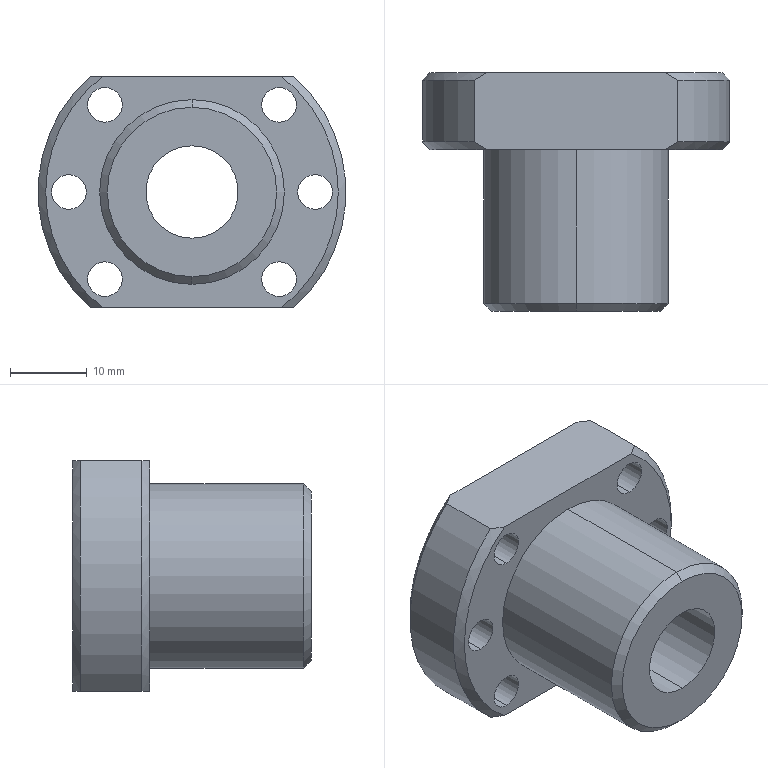Component | SolidWorks | SFS01205Nut--1 | 1 solid | 29 faces | box 40 x 31 x 30 mm | volume 15688 mm3 | cylinder 18 | cone 6 | plane 5 | commonest cylinder face diameters 4.5 x12 24 x2 12 x2 40 x2
build123d program:
from build123d import *

# Parameters (mm, degrees)
CUT_EXTRUDE1_DEPTH = 42.964
SKETCH3_R          = 2.25
CUT_EXTRUDE2_DEPTH = 40.825
CHAMFER1_SIZE      = 1


with BuildPart() as part:
    # Sketch1 → Revolve1 (revolve)
    with BuildSketch(Plane(origin=(0, 0, 0), x_dir=(1, 0, 0), z_dir=(0, 1, 0))):
        Polygon((-31, 6), (-31, 20), (-21, 20), (-21, 12), (0, 12), (0, 6), align=None)
    revolve(axis=Axis((0, 0, 0), (-1, 0, 0)))

    # Sketch2 → Cut-Extrude1 (cut, symmetric)
    with BuildSketch(Plane.ZY.offset(31)):
        Polygon((15, 119.751), (15, 13.229), (15, -13.229), (15, -119.751), (228.045, -119.751), (228.045, 119.751), align=None)
    cut_extrude1 = extrude(amount=CUT_EXTRUDE1_DEPTH, both=True, mode=Mode.SUBTRACT)

    # Mirror1: Cut-Extrude1 across plane
    add(cut_extrude1.mirror(Plane.XY), mode=Mode.SUBTRACT)

    # Sketch3 → Cut-Extrude2 (cut, through all)
    with BuildSketch(Plane.ZY.offset(31)):
        with Locations((-11.314, 11.314)):
            Circle(SKETCH3_R)
        with Locations(Location((11.314, 11.314, 0), (0, 0, 180))):
            Circle(SKETCH3_R)
        with Locations((0, 16)):
            Circle(SKETCH3_R)
        with Locations(Location((0, -16, 0), (0, 0, 180))):
            Circle(SKETCH3_R)
        with Locations((11.314, -11.314)):
            Circle(SKETCH3_R)
        with Locations(Location((-11.314, -11.314, 0), (0, 0, 180))):
            Circle(SKETCH3_R)
    extrude(amount=-CUT_EXTRUDE2_DEPTH, mode=Mode.SUBTRACT)

    # Chamfer1
    chamfer1_edges = [part.edges().sort_by_distance(p)[0] for p in [
        (-21, -20, 0),
        (-31, -20, 0),
        (-21, 20, 0),
        (-31, 20, 0),
        (0, 0, 12),
    ]]
    chamfer(chamfer1_edges, length=CHAMFER1_SIZE)


solid = part.part

# Placed as in the assembly
solid = solid.moved(Location((-109.352, -196.452, -272.475), (0, 0, -90)))
STEP:
#1=COLOUR_RGB('',0.7922,0.8196,0.9333);
#2=FILL_AREA_STYLE_COLOUR('',#1);
#3=FILL_AREA_STYLE('',(#2));
#4=SURFACE_STYLE_FILL_AREA(#3);
#5=SURFACE_SIDE_STYLE('',(#4));
#6=SURFACE_STYLE_USAGE(.BOTH.,#5);
#7=PRESENTATION_STYLE_ASSIGNMENT((#6));
#8=CARTESIAN_POINT('',(-4.305,-7.734,-11.16));
#9=VERTEX_POINT('',#8);
#10=CARTESIAN_POINT('',(-4.305,-7.734,-10.294));
#11=VERTEX_POINT('',#10);
#12=CARTESIAN_POINT('',(-4.305,-7.734,-10.727));
#13=DIRECTION('',(-0.,-1.,0.));
#14=DIRECTION('',(-0.,0.,-1.));
#15=AXIS2_PLACEMENT_3D('',#12,#13,#14);
#16=CIRCLE('',#15,0.4331);
#17=EDGE_CURVE('',#9,#11,#16,.T.);
#18=ORIENTED_EDGE('',*,*,#17,.F.);
#19=CARTESIAN_POINT('',(-4.305,-7.695,-11.2));
#20=VERTEX_POINT('',#19);
#21=CARTESIAN_POINT('',(-4.305,-7.734,-11.16));
#22=DIRECTION('',(-0.,0.7071,-0.7071));
#23=VECTOR('',#22,39.37);
#24=LINE('',#21,#23);
#25=EDGE_CURVE('',#9,#20,#24,.T.);
#26=ORIENTED_EDGE('',*,*,#25,.T.);
#27=CARTESIAN_POINT('',(-4.305,-7.695,-10.255));
#28=VERTEX_POINT('',#27);
#29=CARTESIAN_POINT('',(-4.305,-7.695,-10.727));
#30=DIRECTION('',(0.,1.,-0.));
#31=DIRECTION('',(-0.,0.,-1.));
#32=AXIS2_PLACEMENT_3D('',#29,#30,#31);
#33=CIRCLE('',#32,0.4724);
#34=EDGE_CURVE('',#28,#20,#33,.T.);
#35=ORIENTED_EDGE('',*,*,#34,.F.);
#36=CARTESIAN_POINT('',(-4.305,-7.734,-10.294));
#37=DIRECTION('',(0.,0.7071,0.7071));
#38=VECTOR('',#37,39.37);
#39=LINE('',#36,#38);
#40=EDGE_CURVE('',#11,#28,#39,.T.);
#41=ORIENTED_EDGE('',*,*,#40,.F.);
#42=EDGE_LOOP('',(#18,#26,#35,#41));
#43=FACE_OUTER_BOUND('',#42,.T.);
#44=CARTESIAN_POINT('',(-4.305,-7.734,-10.727));
#45=DIRECTION('',(0.,1.,-0.));
#46=DIRECTION('',(0.,0.,1.));
#47=AXIS2_PLACEMENT_3D('',#44,#45,#46);
#48=CONICAL_SURFACE('',#47,0.4331,0.7854);
#49=ADVANCED_FACE('',(#43),#48,.T.);
#50=CARTESIAN_POINT('',(-4.751,-6.908,-11.084));
#51=VERTEX_POINT('',#50);
#52=CARTESIAN_POINT('',(-4.751,-6.908,-11.261));
#53=VERTEX_POINT('',#52);
#54=CARTESIAN_POINT('',(-4.751,-6.908,-11.173));
#55=DIRECTION('',(-0.,-1.,0.));
#56=DIRECTION('',(-0.,0.,-1.));
#57=AXIS2_PLACEMENT_3D('',#54,#55,#56);
#58=CIRCLE('',#57,0.08858);
#59=EDGE_CURVE('',#51,#53,#58,.T.);
#60=ORIENTED_EDGE('',*,*,#59,.T.);
#61=CARTESIAN_POINT('',(-4.751,-6.514,-11.261));
#62=VERTEX_POINT('',#61);
#63=CARTESIAN_POINT('',(-4.751,-7.734,-11.261));
#64=DIRECTION('',(0.,1.,-0.));
#65=VECTOR('',#64,39.37);
#66=LINE('',#63,#65);
#67=EDGE_CURVE('',#53,#62,#66,.T.);
#68=ORIENTED_EDGE('',*,*,#67,.T.);
#69=CARTESIAN_POINT('',(-4.751,-6.514,-11.084));
#70=VERTEX_POINT('',#69);
#71=CARTESIAN_POINT('',(-4.751,-6.514,-11.173));
#72=DIRECTION('',(0.,1.,-0.));
#73=DIRECTION('',(-0.,0.,-1.));
#74=AXIS2_PLACEMENT_3D('',#71,#72,#73);
#75=CIRCLE('',#74,0.08858);
#76=EDGE_CURVE('',#62,#70,#75,.T.);
#77=ORIENTED_EDGE('',*,*,#76,.T.);
#78=CARTESIAN_POINT('',(-4.751,-7.734,-11.084));
#79=DIRECTION('',(0.,1.,-0.));
#80=VECTOR('',#79,39.37);
#81=LINE('',#78,#80);
#82=EDGE_CURVE('',#51,#70,#81,.T.);
#83=ORIENTED_EDGE('',*,*,#82,.F.);
#84=EDGE_LOOP('',(#60,#68,#77,#83));
#85=FACE_OUTER_BOUND('',#84,.T.);
#86=CARTESIAN_POINT('',(-4.751,-7.734,-11.173));
#87=DIRECTION('',(0.,1.,-0.));
#88=DIRECTION('',(0.,0.,1.));
#89=AXIS2_PLACEMENT_3D('',#86,#87,#88);
#90=CYLINDRICAL_SURFACE('',#89,0.08858);
#91=ADVANCED_FACE('',(#85),#90,.F.);
#92=CARTESIAN_POINT('',(-4.751,-6.908,-10.193));
#93=VERTEX_POINT('',#92);
#94=CARTESIAN_POINT('',(-4.751,-6.908,-10.371));
#95=VERTEX_POINT('',#94);
#96=CARTESIAN_POINT('',(-4.751,-6.908,-10.282));
#97=DIRECTION('',(-0.,-1.,0.));
#98=DIRECTION('',(-0.,0.,-1.));
#99=AXIS2_PLACEMENT_3D('',#96,#97,#98);
#100=CIRCLE('',#99,0.08858);
#101=EDGE_CURVE('',#93,#95,#100,.T.);
#102=ORIENTED_EDGE('',*,*,#101,.T.);
#103=CARTESIAN_POINT('',(-4.751,-6.514,-10.371));
#104=VERTEX_POINT('',#103);
#105=CARTESIAN_POINT('',(-4.751,-7.734,-10.371));
#106=DIRECTION('',(0.,1.,-0.));
#107=VECTOR('',#106,39.37);
#108=LINE('',#105,#107);
#109=EDGE_CURVE('',#95,#104,#108,.T.);
#110=ORIENTED_EDGE('',*,*,#109,.T.);
#111=CARTESIAN_POINT('',(-4.751,-6.514,-10.193));
#112=VERTEX_POINT('',#111);
#113=CARTESIAN_POINT('',(-4.751,-6.514,-10.282));
#114=DIRECTION('',(0.,1.,-0.));
#115=DIRECTION('',(0.,0.,1.));
#116=AXIS2_PLACEMENT_3D('',#113,#114,#115);
#117=CIRCLE('',#116,0.08858);
#118=EDGE_CURVE('',#104,#112,#117,.T.);
#119=ORIENTED_EDGE('',*,*,#118,.T.);
#120=CARTESIAN_POINT('',(-4.751,-7.734,-10.193));
#121=DIRECTION('',(0.,1.,-0.));
#122=VECTOR('',#121,39.37);
#123=LINE('',#120,#122);
#124=EDGE_CURVE('',#93,#112,#123,.T.);
#125=ORIENTED_EDGE('',*,*,#124,.F.);
#126=EDGE_LOOP('',(#102,#110,#119,#125));
#127=FACE_OUTER_BOUND('',#126,.T.);
#128=CARTESIAN_POINT('',(-4.751,-7.734,-10.282));
#129=DIRECTION('',(0.,1.,-0.));
#130=DIRECTION('',(0.,0.,1.));
#131=AXIS2_PLACEMENT_3D('',#128,#129,#130);
#132=CYLINDRICAL_SURFACE('',#131,0.08858);
#133=ADVANCED_FACE('',(#127),#132,.F.);
#134=CARTESIAN_POINT('',(-4.935,-6.908,-10.639));
#135=VERTEX_POINT('',#134);
#136=CARTESIAN_POINT('',(-4.935,-6.908,-10.816));
#137=VERTEX_POINT('',#136);
#138=CARTESIAN_POINT('',(-4.935,-6.908,-10.727));
#139=DIRECTION('',(-0.,-1.,0.));
#140=DIRECTION('',(-0.,0.,-1.));
#141=AXIS2_PLACEMENT_3D('',#138,#139,#140);
#142=CIRCLE('',#141,0.08858);
#143=EDGE_CURVE('',#135,#137,#142,.T.);
#144=ORIENTED_EDGE('',*,*,#143,.T.);
#145=CARTESIAN_POINT('',(-4.935,-6.514,-10.816));
#146=VERTEX_POINT('',#145);
#147=CARTESIAN_POINT('',(-4.935,-7.734,-10.816));
#148=DIRECTION('',(0.,1.,-0.));
#149=VECTOR('',#148,39.37);
#150=LINE('',#147,#149);
#151=EDGE_CURVE('',#137,#146,#150,.T.);
#152=ORIENTED_EDGE('',*,*,#151,.T.);
#153=CARTESIAN_POINT('',(-4.935,-6.514,-10.639));
#154=VERTEX_POINT('',#153);
#155=CARTESIAN_POINT('',(-4.935,-6.514,-10.727));
#156=DIRECTION('',(0.,1.,-0.));
#157=DIRECTION('',(-0.,0.,-1.));
#158=AXIS2_PLACEMENT_3D('',#155,#156,#157);
#159=CIRCLE('',#158,0.08858);
#160=EDGE_CURVE('',#146,#154,#159,.T.);
#161=ORIENTED_EDGE('',*,*,#160,.T.);
#162=CARTESIAN_POINT('',(-4.935,-7.734,-10.639));
#163=DIRECTION('',(0.,1.,-0.));
#164=VECTOR('',#163,39.37);
#165=LINE('',#162,#164);
#166=EDGE_CURVE('',#135,#154,#165,.T.);
#167=ORIENTED_EDGE('',*,*,#166,.F.);
#168=EDGE_LOOP('',(#144,#152,#161,#167));
#169=FACE_OUTER_BOUND('',#168,.T.);
#170=CARTESIAN_POINT('',(-4.935,-7.734,-10.727));
#171=DIRECTION('',(0.,1.,-0.));
#172=DIRECTION('',(0.,0.,1.));
#173=AXIS2_PLACEMENT_3D('',#170,#171,#172);
#174=CYLINDRICAL_SURFACE('',#173,0.08858);
#175=ADVANCED_FACE('',(#169),#174,.F.);
#176=CARTESIAN_POINT('',(-3.675,-6.908,-10.639));
#177=VERTEX_POINT('',#176);
#178=CARTESIAN_POINT('',(-3.675,-6.908,-10.816));
#179=VERTEX_POINT('',#178);
#180=CARTESIAN_POINT('',(-3.675,-6.908,-10.727));
#181=DIRECTION('',(-0.,-1.,0.));
#182=DIRECTION('',(-0.,0.,-1.));
#183=AXIS2_PLACEMENT_3D('',#180,#181,#182);
#184=CIRCLE('',#183,0.08858);
#185=EDGE_CURVE('',#177,#179,#184,.T.);
#186=ORIENTED_EDGE('',*,*,#185,.T.);
#187=CARTESIAN_POINT('',(-3.675,-6.514,-10.816));
#188=VERTEX_POINT('',#187);
#189=CARTESIAN_POINT('',(-3.675,-7.734,-10.816));
#190=DIRECTION('',(0.,1.,-0.));
#191=VECTOR('',#190,39.37);
#192=LINE('',#189,#191);
#193=EDGE_CURVE('',#179,#188,#192,.T.);
#194=ORIENTED_EDGE('',*,*,#193,.T.);
#195=CARTESIAN_POINT('',(-3.675,-6.514,-10.639));
#196=VERTEX_POINT('',#195);
#197=CARTESIAN_POINT('',(-3.675,-6.514,-10.727));
#198=DIRECTION('',(0.,1.,-0.));
#199=DIRECTION('',(0.,0.,1.));
#200=AXIS2_PLACEMENT_3D('',#197,#198,#199);
#201=CIRCLE('',#200,0.08858);
#202=EDGE_CURVE('',#188,#196,#201,.T.);
#203=ORIENTED_EDGE('',*,*,#202,.T.);
#204=CARTESIAN_POINT('',(-3.675,-7.734,-10.639));
#205=DIRECTION('',(0.,1.,-0.));
#206=VECTOR('',#205,39.37);
#207=LINE('',#204,#206);
#208=EDGE_CURVE('',#177,#196,#207,.T.);
#209=ORIENTED_EDGE('',*,*,#208,.F.);
#210=EDGE_LOOP('',(#186,#194,#203,#209));
#211=FACE_OUTER_BOUND('',#210,.T.);
#212=CARTESIAN_POINT('',(-3.675,-7.734,-10.727));
#213=DIRECTION('',(0.,1.,-0.));
#214=DIRECTION('',(0.,0.,1.));
#215=AXIS2_PLACEMENT_3D('',#212,#213,#214);
#216=CYLINDRICAL_SURFACE('',#215,0.08858);
#217=ADVANCED_FACE('',(#211),#216,.F.);
#218=CARTESIAN_POINT('',(-3.86,-6.908,-10.193));
#219=VERTEX_POINT('',#218);
#220=CARTESIAN_POINT('',(-3.86,-6.908,-10.371));
#221=VERTEX_POINT('',#220);
#222=CARTESIAN_POINT('',(-3.86,-6.908,-10.282));
#223=DIRECTION('',(-0.,-1.,0.));
#224=DIRECTION('',(-0.,0.,-1.));
#225=AXIS2_PLACEMENT_3D('',#222,#223,#224);
#226=CIRCLE('',#225,0.08858);
#227=EDGE_CURVE('',#219,#221,#226,.T.);
#228=ORIENTED_EDGE('',*,*,#227,.T.);
#229=CARTESIAN_POINT('',(-3.86,-6.514,-10.371));
#230=VERTEX_POINT('',#229);
#231=CARTESIAN_POINT('',(-3.86,-7.734,-10.371));
#232=DIRECTION('',(0.,1.,-0.));
#233=VECTOR('',#232,39.37);
#234=LINE('',#231,#233);
#235=EDGE_CURVE('',#221,#230,#234,.T.);
#236=ORIENTED_EDGE('',*,*,#235,.T.);
#237=CARTESIAN_POINT('',(-3.86,-6.514,-10.193));
#238=VERTEX_POINT('',#237);
#239=CARTESIAN_POINT('',(-3.86,-6.514,-10.282));
#240=DIRECTION('',(0.,1.,-0.));
#241=DIRECTION('',(-0.,0.,-1.));
#242=AXIS2_PLACEMENT_3D('',#239,#240,#241);
#243=CIRCLE('',#242,0.08858);
#244=EDGE_CURVE('',#230,#238,#243,.T.);
#245=ORIENTED_EDGE('',*,*,#244,.T.);
#246=CARTESIAN_POINT('',(-3.86,-7.734,-10.193));
#247=DIRECTION('',(0.,1.,-0.));
#248=VECTOR('',#247,39.37);
#249=LINE('',#246,#248);
#250=EDGE_CURVE('',#219,#238,#249,.T.);
#251=ORIENTED_EDGE('',*,*,#250,.F.);
#252=EDGE_LOOP('',(#228,#236,#245,#251));
#253=FACE_OUTER_BOUND('',#252,.T.);
#254=CARTESIAN_POINT('',(-3.86,-7.734,-10.282));
#255=DIRECTION('',(0.,1.,-0.));
#256=DIRECTION('',(0.,0.,1.));
#257=AXIS2_PLACEMENT_3D('',#254,#255,#256);
#258=CYLINDRICAL_SURFACE('',#257,0.08858);
#259=ADVANCED_FACE('',(#253),#258,.F.);
#260=CARTESIAN_POINT('',(-3.86,-6.908,-11.084));
#261=VERTEX_POINT('',#260);
#262=CARTESIAN_POINT('',(-3.86,-6.908,-11.261));
#263=VERTEX_POINT('',#262);
#264=CARTESIAN_POINT('',(-3.86,-6.908,-11.173));
#265=DIRECTION('',(-0.,-1.,0.));
#266=DIRECTION('',(-0.,0.,-1.));
#267=AXIS2_PLACEMENT_3D('',#264,#265,#266);
#268=CIRCLE('',#267,0.08858);
#269=EDGE_CURVE('',#261,#263,#268,.T.);
#270=ORIENTED_EDGE('',*,*,#269,.T.);
#271=CARTESIAN_POINT('',(-3.86,-6.514,-11.261));
#272=VERTEX_POINT('',#271);
#273=CARTESIAN_POINT('',(-3.86,-7.734,-11.261));
#274=DIRECTION('',(0.,1.,-0.));
#275=VECTOR('',#274,39.37);
#276=LINE('',#273,#275);
#277=EDGE_CURVE('',#263,#272,#276,.T.);
#278=ORIENTED_EDGE('',*,*,#277,.T.);
#279=CARTESIAN_POINT('',(-3.86,-6.514,-11.084));
#280=VERTEX_POINT('',#279);
#281=CARTESIAN_POINT('',(-3.86,-6.514,-11.173));
#282=DIRECTION('',(0.,1.,-0.));
#283=DIRECTION('',(0.,0.,1.));
#284=AXIS2_PLACEMENT_3D('',#281,#282,#283);
#285=CIRCLE('',#284,0.08858);
#286=EDGE_CURVE('',#272,#280,#285,.T.);
#287=ORIENTED_EDGE('',*,*,#286,.T.);
#288=CARTESIAN_POINT('',(-3.86,-7.734,-11.084));
#289=DIRECTION('',(0.,1.,-0.));
#290=VECTOR('',#289,39.37);
#291=LINE('',#288,#290);
#292=EDGE_CURVE('',#261,#280,#291,.T.);
#293=ORIENTED_EDGE('',*,*,#292,.F.);
#294=EDGE_LOOP('',(#270,#278,#287,#293));
#295=FACE_OUTER_BOUND('',#294,.T.);
#296=CARTESIAN_POINT('',(-3.86,-7.734,-11.173));
#297=DIRECTION('',(0.,1.,-0.));
#298=DIRECTION('',(0.,0.,1.));
#299=AXIS2_PLACEMENT_3D('',#296,#297,#298);
#300=CYLINDRICAL_SURFACE('',#299,0.08858);
#301=ADVANCED_FACE('',(#295),#300,.F.);
#302=CARTESIAN_POINT('',(-4.305,-6.908,-11.2));
#303=VERTEX_POINT('',#302);
#304=CARTESIAN_POINT('',(-4.305,-6.908,-10.255));
#305=VERTEX_POINT('',#304);
#306=CARTESIAN_POINT('',(-4.305,-6.908,-10.727));
#307=DIRECTION('',(-0.,-1.,0.));
#308=DIRECTION('',(-0.,0.,-1.));
#309=AXIS2_PLACEMENT_3D('',#306,#307,#308);
#310=CIRCLE('',#309,0.4724);
#311=EDGE_CURVE('',#303,#305,#310,.T.);
#312=ORIENTED_EDGE('',*,*,#311,.T.);
#313=CARTESIAN_POINT('',(-4.305,-7.734,-10.255));
#314=DIRECTION('',(-0.,-1.,0.));
#315=VECTOR('',#314,39.37);
#316=LINE('',#313,#315);
#317=EDGE_CURVE('',#305,#28,#316,.T.);
#318=ORIENTED_EDGE('',*,*,#317,.T.);
#319=ORIENTED_EDGE('',*,*,#34,.T.);
#320=CARTESIAN_POINT('',(-4.305,-7.734,-11.2));
#321=DIRECTION('',(-0.,-1.,0.));
#322=VECTOR('',#321,39.37);
#323=LINE('',#320,#322);
#324=EDGE_CURVE('',#303,#20,#323,.T.);
#325=ORIENTED_EDGE('',*,*,#324,.F.);
#326=EDGE_LOOP('',(#312,#318,#319,#325));
#327=FACE_OUTER_BOUND('',#326,.T.);
#328=CARTESIAN_POINT('',(-4.305,-7.734,-10.727));
#329=DIRECTION('',(-0.,-1.,0.));
#330=DIRECTION('',(-0.,0.,-1.));
#331=AXIS2_PLACEMENT_3D('',#328,#329,#330);
#332=CYLINDRICAL_SURFACE('',#331,0.4724);
#333=ADVANCED_FACE('',(#327),#332,.T.);
#334=CARTESIAN_POINT('',(-4.305,-6.514,-10.491));
#335=VERTEX_POINT('',#334);
#336=CARTESIAN_POINT('',(-4.305,-6.514,-10.964));
#337=VERTEX_POINT('',#336);
#338=CARTESIAN_POINT('',(-4.305,-6.514,-10.727));
#339=DIRECTION('',(-0.,-1.,0.));
#340=DIRECTION('',(-0.,0.,-1.));
#341=AXIS2_PLACEMENT_3D('',#338,#339,#340);
#342=CIRCLE('',#341,0.2362);
#343=EDGE_CURVE('',#335,#337,#342,.T.);
#344=ORIENTED_EDGE('',*,*,#343,.F.);
#345=CARTESIAN_POINT('',(-4.305,-7.734,-10.491));
#346=VERTEX_POINT('',#345);
#347=CARTESIAN_POINT('',(-4.305,-7.734,-10.491));
#348=DIRECTION('',(-0.,-1.,0.));
#349=VECTOR('',#348,39.37);
#350=LINE('',#347,#349);
#351=EDGE_CURVE('',#335,#346,#350,.T.);
#352=ORIENTED_EDGE('',*,*,#351,.T.);
#353=CARTESIAN_POINT('',(-4.305,-7.734,-10.964));
#354=VERTEX_POINT('',#353);
#355=CARTESIAN_POINT('',(-4.305,-7.734,-10.727));
#356=DIRECTION('',(-0.,-1.,0.));
#357=DIRECTION('',(-0.,0.,-1.));
#358=AXIS2_PLACEMENT_3D('',#355,#356,#357);
#359=CIRCLE('',#358,0.2362);
#360=EDGE_CURVE('',#346,#354,#359,.T.);
#361=ORIENTED_EDGE('',*,*,#360,.T.);
#362=CARTESIAN_POINT('',(-4.305,-7.734,-10.964));
#363=DIRECTION('',(-0.,-1.,0.));
#364=VECTOR('',#363,39.37);
#365=LINE('',#362,#364);
#366=EDGE_CURVE('',#337,#354,#365,.T.);
#367=ORIENTED_EDGE('',*,*,#366,.F.);
#368=EDGE_LOOP('',(#344,#352,#361,#367));
#369=FACE_OUTER_BOUND('',#368,.T.);
#370=CARTESIAN_POINT('',(-4.305,-7.734,-10.727));
#371=DIRECTION('',(-0.,-1.,0.));
#372=DIRECTION('',(-0.,0.,-1.));
#373=AXIS2_PLACEMENT_3D('',#370,#371,#372);
#374=CYLINDRICAL_SURFACE('',#373,0.2362);
#375=ADVANCED_FACE('',(#369),#374,.F.);
#376=CARTESIAN_POINT('',(-4.826,-6.553,-10.137));
#377=VERTEX_POINT('',#376);
#378=CARTESIAN_POINT('',(-4.826,-6.868,-10.137));
#379=VERTEX_POINT('',#378);
#380=CARTESIAN_POINT('',(-4.826,-1.814,-10.137));
#381=DIRECTION('',(-0.,-1.,0.));
#382=VECTOR('',#381,39.37);
#383=LINE('',#380,#382);
#384=EDGE_CURVE('',#377,#379,#383,.T.);
#385=ORIENTED_EDGE('',*,*,#384,.F.);
#386=CARTESIAN_POINT('',(-4.826,-6.553,-11.318));
#387=VERTEX_POINT('',#386);
#388=CARTESIAN_POINT('',(-4.305,-6.553,-10.727));
#389=DIRECTION('',(-0.,-1.,0.));
#390=DIRECTION('',(0.,0.,1.));
#391=AXIS2_PLACEMENT_3D('',#388,#389,#390);
#392=CIRCLE('',#391,0.7874);
#393=EDGE_CURVE('',#377,#387,#392,.T.);
#394=ORIENTED_EDGE('',*,*,#393,.T.);
#395=CARTESIAN_POINT('',(-4.826,-6.868,-11.318));
#396=VERTEX_POINT('',#395);
#397=CARTESIAN_POINT('',(-4.826,-3.486,-11.318));
#398=DIRECTION('',(0.,-1.,0.));
#399=VECTOR('',#398,39.37);
#400=LINE('',#397,#399);
#401=EDGE_CURVE('',#387,#396,#400,.T.);
#402=ORIENTED_EDGE('',*,*,#401,.T.);
#403=CARTESIAN_POINT('',(-4.305,-6.868,-10.727));
#404=DIRECTION('',(0.,1.,-0.));
#405=DIRECTION('',(-0.,0.,-1.));
#406=AXIS2_PLACEMENT_3D('',#403,#404,#405);
#407=CIRCLE('',#406,0.7874);
#408=EDGE_CURVE('',#396,#379,#407,.T.);
#409=ORIENTED_EDGE('',*,*,#408,.T.);
#410=EDGE_LOOP('',(#385,#394,#402,#409));
#411=FACE_OUTER_BOUND('',#410,.T.);
#412=CARTESIAN_POINT('',(-4.305,-7.734,-10.727));
#413=DIRECTION('',(-0.,-1.,0.));
#414=DIRECTION('',(-0.,0.,-1.));
#415=AXIS2_PLACEMENT_3D('',#412,#413,#414);
#416=CYLINDRICAL_SURFACE('',#415,0.7874);
#417=ADVANCED_FACE('',(#411),#416,.T.);
#418=CARTESIAN_POINT('',(-4.751,-6.514,-11.173));
#419=DIRECTION('',(0.,1.,-0.));
#420=DIRECTION('',(-0.,0.,-1.));
#421=AXIS2_PLACEMENT_3D('',#418,#419,#420);
#422=CIRCLE('',#421,0.08858);
#423=EDGE_CURVE('',#70,#62,#422,.T.);
#424=ORIENTED_EDGE('',*,*,#423,.F.);
#425=ORIENTED_EDGE('',*,*,#76,.F.);
#426=EDGE_LOOP('',(#424,#425));
#427=FACE_BOUND('',#426,.T.);
#428=CARTESIAN_POINT('',(-4.751,-6.514,-10.282));
#429=DIRECTION('',(0.,1.,-0.));
#430=DIRECTION('',(0.,0.,1.));
#431=AXIS2_PLACEMENT_3D('',#428,#429,#430);
#432=CIRCLE('',#431,0.08858);
#433=EDGE_CURVE('',#112,#104,#432,.T.);
#434=ORIENTED_EDGE('',*,*,#433,.F.);
#435=ORIENTED_EDGE('',*,*,#118,.F.);
#436=EDGE_LOOP('',(#434,#435));
#437=FACE_BOUND('',#436,.T.);
#438=CARTESIAN_POINT('',(-4.935,-6.514,-10.727));
#439=DIRECTION('',(0.,1.,-0.));
#440=DIRECTION('',(-0.,0.,-1.));
#441=AXIS2_PLACEMENT_3D('',#438,#439,#440);
#442=CIRCLE('',#441,0.08858);
#443=EDGE_CURVE('',#154,#146,#442,.T.);
#444=ORIENTED_EDGE('',*,*,#443,.F.);
#445=ORIENTED_EDGE('',*,*,#160,.F.);
#446=EDGE_LOOP('',(#444,#445));
#447=FACE_BOUND('',#446,.T.);
#448=CARTESIAN_POINT('',(-3.675,-6.514,-10.727));
#449=DIRECTION('',(0.,1.,-0.));
#450=DIRECTION('',(0.,0.,1.));
#451=AXIS2_PLACEMENT_3D('',#448,#449,#450);
#452=CIRCLE('',#451,0.08858);
#453=EDGE_CURVE('',#196,#188,#452,.T.);
#454=ORIENTED_EDGE('',*,*,#453,.F.);
#455=ORIENTED_EDGE('',*,*,#202,.F.);
#456=EDGE_LOOP('',(#454,#455));
#457=FACE_BOUND('',#456,.T.);
#458=CARTESIAN_POINT('',(-3.86,-6.514,-10.282));
#459=DIRECTION('',(0.,1.,-0.));
#460=DIRECTION('',(-0.,0.,-1.));
#461=AXIS2_PLACEMENT_3D('',#458,#459,#460);
#462=CIRCLE('',#461,0.08858);
#463=EDGE_CURVE('',#238,#230,#462,.T.);
#464=ORIENTED_EDGE('',*,*,#463,.F.);
#465=ORIENTED_EDGE('',*,*,#244,.F.);
#466=EDGE_LOOP('',(#464,#465));
#467=FACE_BOUND('',#466,.T.);
#468=CARTESIAN_POINT('',(-3.86,-6.514,-11.173));
#469=DIRECTION('',(0.,1.,-0.));
#470=DIRECTION('',(0.,0.,1.));
#471=AXIS2_PLACEMENT_3D('',#468,#469,#470);
#472=CIRCLE('',#471,0.08858);
#473=EDGE_CURVE('',#280,#272,#472,.T.);
#474=ORIENTED_EDGE('',*,*,#473,.F.);
#475=ORIENTED_EDGE('',*,*,#286,.F.);
#476=EDGE_LOOP('',(#474,#475));
#477=FACE_BOUND('',#476,.T.);
#478=CARTESIAN_POINT('',(-4.764,-6.514,-10.137));
#479=VERTEX_POINT('',#478);
#480=CARTESIAN_POINT('',(-3.846,-6.514,-10.137));
#481=VERTEX_POINT('',#480);
#482=CARTESIAN_POINT('',(-4.305,-6.514,-10.137));
#483=DIRECTION('',(1.,-0.,-0.));
#484=VECTOR('',#483,39.37);
#485=LINE('',#482,#484);
#486=EDGE_CURVE('',#479,#481,#485,.T.);
#487=ORIENTED_EDGE('',*,*,#486,.T.);
#488=CARTESIAN_POINT('',(-3.846,-6.514,-11.318));
#489=VERTEX_POINT('',#488);
#490=CARTESIAN_POINT('',(-4.305,-6.514,-10.727));
#491=DIRECTION('',(0.,1.,-0.));
#492=DIRECTION('',(0.,0.,1.));
#493=AXIS2_PLACEMENT_3D('',#490,#491,#492);
#494=CIRCLE('',#493,0.748);
#495=EDGE_CURVE('',#481,#489,#494,.T.);
#496=ORIENTED_EDGE('',*,*,#495,.T.);
#497=CARTESIAN_POINT('',(-4.764,-6.514,-11.318));
#498=VERTEX_POINT('',#497);
#499=CARTESIAN_POINT('',(-4.305,-6.514,-11.318));
#500=DIRECTION('',(1.,-0.,-0.));
#501=VECTOR('',#500,39.37);
#502=LINE('',#499,#501);
#503=EDGE_CURVE('',#498,#489,#502,.T.);
#504=ORIENTED_EDGE('',*,*,#503,.F.);
#505=CARTESIAN_POINT('',(-4.305,-6.514,-10.727));
#506=DIRECTION('',(0.,1.,-0.));
#507=DIRECTION('',(0.,0.,1.));
#508=AXIS2_PLACEMENT_3D('',#505,#506,#507);
#509=CIRCLE('',#508,0.748);
#510=EDGE_CURVE('',#498,#479,#509,.T.);
#511=ORIENTED_EDGE('',*,*,#510,.T.);
#512=EDGE_LOOP('',(#487,#496,#504,#511));
#513=FACE_OUTER_BOUND('',#512,.T.);
#514=CARTESIAN_POINT('',(-4.305,-6.514,-10.727));
#515=DIRECTION('',(-0.,-1.,0.));
#516=DIRECTION('',(-0.,0.,-1.));
#517=AXIS2_PLACEMENT_3D('',#514,#515,#516);
#518=CIRCLE('',#517,0.2362);
#519=EDGE_CURVE('',#337,#335,#518,.T.);
#520=ORIENTED_EDGE('',*,*,#519,.T.);
#521=ORIENTED_EDGE('',*,*,#343,.T.);
#522=EDGE_LOOP('',(#520,#521));
#523=FACE_BOUND('',#522,.T.);
#524=CARTESIAN_POINT('',(-4.305,-6.514,-10.964));
#525=DIRECTION('',(0.,1.,-0.));
#526=DIRECTION('',(0.,0.,1.));
#527=AXIS2_PLACEMENT_3D('',#524,#525,#526);
#528=PLANE('',#527);
#529=ADVANCED_FACE('',(#427,#437,#447,#457,#467,#477,#513,#523),#528,.T.);
#530=CARTESIAN_POINT('',(-3.784,-6.553,-10.137));
#531=VERTEX_POINT('',#530);
#532=CARTESIAN_POINT('',(-3.784,-6.868,-10.137));
#533=VERTEX_POINT('',#532);
#534=CARTESIAN_POINT('',(-3.784,-1.814,-10.137));
#535=DIRECTION('',(-0.,-1.,0.));
#536=VECTOR('',#535,39.37);
#537=LINE('',#534,#536);
#538=EDGE_CURVE('',#531,#533,#537,.T.);
#539=ORIENTED_EDGE('',*,*,#538,.T.);
#540=CARTESIAN_POINT('',(-3.784,-6.868,-11.318));
#541=VERTEX_POINT('',#540);
#542=CARTESIAN_POINT('',(-4.305,-6.868,-10.727));
#543=DIRECTION('',(0.,1.,-0.));
#544=DIRECTION('',(-0.,0.,-1.));
#545=AXIS2_PLACEMENT_3D('',#542,#543,#544);
#546=CIRCLE('',#545,0.7874);
#547=EDGE_CURVE('',#533,#541,#546,.T.);
#548=ORIENTED_EDGE('',*,*,#547,.T.);
#549=CARTESIAN_POINT('',(-3.784,-6.553,-11.318));
#550=VERTEX_POINT('',#549);
#551=CARTESIAN_POINT('',(-3.784,-3.486,-11.318));
#552=DIRECTION('',(0.,-1.,0.));
#553=VECTOR('',#552,39.37);
#554=LINE('',#551,#553);
#555=EDGE_CURVE('',#550,#541,#554,.T.);
#556=ORIENTED_EDGE('',*,*,#555,.F.);
#557=CARTESIAN_POINT('',(-4.305,-6.553,-10.727));
#558=DIRECTION('',(-0.,-1.,0.));
#559=DIRECTION('',(0.,0.,1.));
#560=AXIS2_PLACEMENT_3D('',#557,#558,#559);
#561=CIRCLE('',#560,0.7874);
#562=EDGE_CURVE('',#550,#531,#561,.T.);
#563=ORIENTED_EDGE('',*,*,#562,.T.);
#564=EDGE_LOOP('',(#539,#548,#556,#563));
#565=FACE_OUTER_BOUND('',#564,.T.);
#566=CARTESIAN_POINT('',(-4.305,-7.734,-10.727));
#567=DIRECTION('',(-0.,-1.,0.));
#568=DIRECTION('',(-0.,0.,-1.));
#569=AXIS2_PLACEMENT_3D('',#566,#567,#568);
#570=CYLINDRICAL_SURFACE('',#569,0.7874);
#571=ADVANCED_FACE('',(#565),#570,.T.);
#572=ORIENTED_EDGE('',*,*,#59,.F.);
#573=CARTESIAN_POINT('',(-4.751,-6.908,-11.173));
#574=DIRECTION('',(-0.,-1.,0.));
#575=DIRECTION('',(-0.,0.,-1.));
#576=AXIS2_PLACEMENT_3D('',#573,#574,#575);
#577=CIRCLE('',#576,0.08858);
#578=EDGE_CURVE('',#53,#51,#577,.T.);
#579=ORIENTED_EDGE('',*,*,#578,.F.);
#580=EDGE_LOOP('',(#572,#579));
#581=FACE_BOUND('',#580,.T.);
#582=ORIENTED_EDGE('',*,*,#101,.F.);
#583=CARTESIAN_POINT('',(-4.751,-6.908,-10.282));
#584=DIRECTION('',(-0.,-1.,0.));
#585=DIRECTION('',(-0.,0.,-1.));
#586=AXIS2_PLACEMENT_3D('',#583,#584,#585);
#587=CIRCLE('',#586,0.08858);
#588=EDGE_CURVE('',#95,#93,#587,.T.);
#589=ORIENTED_EDGE('',*,*,#588,.F.);
#590=EDGE_LOOP('',(#582,#589));
#591=FACE_BOUND('',#590,.T.);
#592=ORIENTED_EDGE('',*,*,#143,.F.);
#593=CARTESIAN_POINT('',(-4.935,-6.908,-10.727));
#594=DIRECTION('',(-0.,-1.,0.));
#595=DIRECTION('',(-0.,0.,-1.));
#596=AXIS2_PLACEMENT_3D('',#593,#594,#595);
#597=CIRCLE('',#596,0.08858);
#598=EDGE_CURVE('',#137,#135,#597,.T.);
#599=ORIENTED_EDGE('',*,*,#598,.F.);
#600=EDGE_LOOP('',(#592,#599));
#601=FACE_BOUND('',#600,.T.);
#602=ORIENTED_EDGE('',*,*,#185,.F.);
#603=CARTESIAN_POINT('',(-3.675,-6.908,-10.727));
#604=DIRECTION('',(-0.,-1.,0.));
#605=DIRECTION('',(-0.,0.,-1.));
#606=AXIS2_PLACEMENT_3D('',#603,#604,#605);
#607=CIRCLE('',#606,0.08858);
#608=EDGE_CURVE('',#179,#177,#607,.T.);
#609=ORIENTED_EDGE('',*,*,#608,.F.);
#610=EDGE_LOOP('',(#602,#609));
#611=FACE_BOUND('',#610,.T.);
#612=ORIENTED_EDGE('',*,*,#227,.F.);
#613=CARTESIAN_POINT('',(-3.86,-6.908,-10.282));
#614=DIRECTION('',(-0.,-1.,0.));
#615=DIRECTION('',(-0.,0.,-1.));
#616=AXIS2_PLACEMENT_3D('',#613,#614,#615);
#617=CIRCLE('',#616,0.08858);
#618=EDGE_CURVE('',#221,#219,#617,.T.);
#619=ORIENTED_EDGE('',*,*,#618,.F.);
#620=EDGE_LOOP('',(#612,#619));
#621=FACE_BOUND('',#620,.T.);
#622=ORIENTED_EDGE('',*,*,#269,.F.);
#623=CARTESIAN_POINT('',(-3.86,-6.908,-11.173));
#624=DIRECTION('',(-0.,-1.,0.));
#625=DIRECTION('',(-0.,0.,-1.));
#626=AXIS2_PLACEMENT_3D('',#623,#624,#625);
#627=CIRCLE('',#626,0.08858);
#628=EDGE_CURVE('',#263,#261,#627,.T.);
#629=ORIENTED_EDGE('',*,*,#628,.F.);
#630=EDGE_LOOP('',(#622,#629));
#631=FACE_BOUND('',#630,.T.);
#632=CARTESIAN_POINT('',(-3.846,-6.908,-11.318));
#633=VERTEX_POINT('',#632);
#634=CARTESIAN_POINT('',(-4.764,-6.908,-11.318));
#635=VERTEX_POINT('',#634);
#636=CARTESIAN_POINT('',(-4.305,-6.908,-11.318));
#637=DIRECTION('',(-1.,0.,0.));
#638=VECTOR('',#637,39.37);
#639=LINE('',#636,#638);
#640=EDGE_CURVE('',#633,#635,#639,.T.);
#641=ORIENTED_EDGE('',*,*,#640,.F.);
#642=CARTESIAN_POINT('',(-3.846,-6.908,-10.137));
#643=VERTEX_POINT('',#642);
#644=CARTESIAN_POINT('',(-4.305,-6.908,-10.727));
#645=DIRECTION('',(-0.,-1.,0.));
#646=DIRECTION('',(-0.,0.,-1.));
#647=AXIS2_PLACEMENT_3D('',#644,#645,#646);
#648=CIRCLE('',#647,0.748);
#649=EDGE_CURVE('',#633,#643,#648,.T.);
#650=ORIENTED_EDGE('',*,*,#649,.T.);
#651=CARTESIAN_POINT('',(-4.764,-6.908,-10.137));
#652=VERTEX_POINT('',#651);
#653=CARTESIAN_POINT('',(-4.305,-6.908,-10.137));
#654=DIRECTION('',(-1.,0.,0.));
#655=VECTOR('',#654,39.37);
#656=LINE('',#653,#655);
#657=EDGE_CURVE('',#643,#652,#656,.T.);
#658=ORIENTED_EDGE('',*,*,#657,.T.);
#659=CARTESIAN_POINT('',(-4.305,-6.908,-10.727));
#660=DIRECTION('',(-0.,-1.,0.));
#661=DIRECTION('',(-0.,0.,-1.));
#662=AXIS2_PLACEMENT_3D('',#659,#660,#661);
#663=CIRCLE('',#662,0.748);
#664=EDGE_CURVE('',#652,#635,#663,.T.);
#665=ORIENTED_EDGE('',*,*,#664,.T.);
#666=EDGE_LOOP('',(#641,#650,#658,#665));
#667=FACE_OUTER_BOUND('',#666,.T.);
#668=ORIENTED_EDGE('',*,*,#311,.F.);
#669=CARTESIAN_POINT('',(-4.305,-6.908,-10.727));
#670=DIRECTION('',(-0.,-1.,0.));
#671=DIRECTION('',(-0.,0.,-1.));
#672=AXIS2_PLACEMENT_3D('',#669,#670,#671);
#673=CIRCLE('',#672,0.4724);
#674=EDGE_CURVE('',#305,#303,#673,.T.);
#675=ORIENTED_EDGE('',*,*,#674,.F.);
#676=EDGE_LOOP('',(#668,#675));
#677=FACE_BOUND('',#676,.T.);
#678=CARTESIAN_POINT('',(-4.305,-6.908,-11.515));
#679=DIRECTION('',(-0.,-1.,0.));
#680=DIRECTION('',(-0.,-0.,-1.));
#681=AXIS2_PLACEMENT_3D('',#678,#679,#680);
#682=PLANE('',#681);
#683=ADVANCED_FACE('',(#581,#591,#601,#611,#621,#631,#667,#677),#682,.T.);
#684=ORIENTED_EDGE('',*,*,#351,.F.);
#685=ORIENTED_EDGE('',*,*,#519,.F.);
#686=ORIENTED_EDGE('',*,*,#366,.T.);
#687=CARTESIAN_POINT('',(-4.305,-7.734,-10.727));
#688=DIRECTION('',(-0.,-1.,0.));
#689=DIRECTION('',(-0.,0.,-1.));
#690=AXIS2_PLACEMENT_3D('',#687,#688,#689);
#691=CIRCLE('',#690,0.2362);
#692=EDGE_CURVE('',#354,#346,#691,.T.);
#693=ORIENTED_EDGE('',*,*,#692,.T.);
#694=EDGE_LOOP('',(#684,#685,#686,#693));
#695=FACE_OUTER_BOUND('',#694,.T.);
#696=CARTESIAN_POINT('',(-4.305,-7.734,-10.727));
#697=DIRECTION('',(-0.,-1.,0.));
#698=DIRECTION('',(-0.,0.,-1.));
#699=AXIS2_PLACEMENT_3D('',#696,#697,#698);
#700=CYLINDRICAL_SURFACE('',#699,0.2362);
#701=ADVANCED_FACE('',(#695),#700,.F.);
#702=ORIENTED_EDGE('',*,*,#317,.F.);
#703=ORIENTED_EDGE('',*,*,#674,.T.);
#704=ORIENTED_EDGE('',*,*,#324,.T.);
#705=CARTESIAN_POINT('',(-4.305,-7.695,-10.727));
#706=DIRECTION('',(0.,1.,-0.));
#707=DIRECTION('',(-0.,0.,-1.));
#708=AXIS2_PLACEMENT_3D('',#705,#706,#707);
#709=CIRCLE('',#708,0.4724);
#710=EDGE_CURVE('',#20,#28,#709,.T.);
#711=ORIENTED_EDGE('',*,*,#710,.T.);
#712=EDGE_LOOP('',(#702,#703,#704,#711));
#713=FACE_OUTER_BOUND('',#712,.T.);
#714=CARTESIAN_POINT('',(-4.305,-7.734,-10.727));
#715=DIRECTION('',(-0.,-1.,0.));
#716=DIRECTION('',(-0.,0.,-1.));
#717=AXIS2_PLACEMENT_3D('',#714,#715,#716);
#718=CYLINDRICAL_SURFACE('',#717,0.4724);
#719=ADVANCED_FACE('',(#713),#718,.T.);
#720=CARTESIAN_POINT('',(-4.305,-7.734,-10.727));
#721=DIRECTION('',(-0.,-1.,0.));
#722=DIRECTION('',(-0.,0.,-1.));
#723=AXIS2_PLACEMENT_3D('',#720,#721,#722);
#724=CIRCLE('',#723,0.4331);
#725=EDGE_CURVE('',#11,#9,#724,.T.);
#726=ORIENTED_EDGE('',*,*,#725,.T.);
#727=ORIENTED_EDGE('',*,*,#17,.T.);
#728=EDGE_LOOP('',(#726,#727));
#729=FACE_OUTER_BOUND('',#728,.T.);
#730=ORIENTED_EDGE('',*,*,#692,.F.);
#731=ORIENTED_EDGE('',*,*,#360,.F.);
#732=EDGE_LOOP('',(#730,#731));
#733=FACE_BOUND('',#732,.T.);
#734=CARTESIAN_POINT('',(-4.305,-7.734,-11.2));
#735=DIRECTION('',(-0.,-1.,0.));
#736=DIRECTION('',(-0.,-0.,-1.));
#737=AXIS2_PLACEMENT_3D('',#734,#735,#736);
#738=PLANE('',#737);
#739=ADVANCED_FACE('',(#729,#733),#738,.T.);
#740=ORIENTED_EDGE('',*,*,#657,.F.);
#741=CARTESIAN_POINT('',(-3.846,-6.908,-10.137));
#742=CARTESIAN_POINT('',(-3.825,-6.895,-10.137));
#743=CARTESIAN_POINT('',(-3.805,-6.882,-10.137));
#744=CARTESIAN_POINT('',(-3.784,-6.868,-10.137));
#745=B_SPLINE_CURVE_WITH_KNOTS('',3,(#741,#742,#743,#744),.UNSPECIFIED.,.F.,.F.,(4,4),(0.,0.001859),.UNSPECIFIED.);
#746=EDGE_CURVE('',#643,#533,#745,.T.);
#747=ORIENTED_EDGE('',*,*,#746,.T.);
#748=ORIENTED_EDGE('',*,*,#538,.F.);
#749=CARTESIAN_POINT('',(-3.784,-6.553,-10.137));
#750=CARTESIAN_POINT('',(-3.805,-6.54,-10.137));
#751=CARTESIAN_POINT('',(-3.825,-6.527,-10.137));
#752=CARTESIAN_POINT('',(-3.846,-6.514,-10.137));
#753=B_SPLINE_CURVE_WITH_KNOTS('',3,(#749,#750,#751,#752),.UNSPECIFIED.,.F.,.F.,(4,4),(0.,0.001859),.UNSPECIFIED.);
#754=EDGE_CURVE('',#531,#481,#753,.T.);
#755=ORIENTED_EDGE('',*,*,#754,.T.);
#756=ORIENTED_EDGE('',*,*,#486,.F.);
#757=CARTESIAN_POINT('',(-4.764,-6.514,-10.137));
#758=CARTESIAN_POINT('',(-4.785,-6.527,-10.137));
#759=CARTESIAN_POINT('',(-4.806,-6.54,-10.137));
#760=CARTESIAN_POINT('',(-4.826,-6.553,-10.137));
#761=B_SPLINE_CURVE_WITH_KNOTS('',3,(#757,#758,#759,#760),.UNSPECIFIED.,.F.,.F.,(4,4),(0.,0.001859),.UNSPECIFIED.);
#762=EDGE_CURVE('',#479,#377,#761,.T.);
#763=ORIENTED_EDGE('',*,*,#762,.T.);
#764=ORIENTED_EDGE('',*,*,#384,.T.);
#765=CARTESIAN_POINT('',(-4.826,-6.868,-10.137));
#766=CARTESIAN_POINT('',(-4.806,-6.882,-10.137));
#767=CARTESIAN_POINT('',(-4.785,-6.895,-10.137));
#768=CARTESIAN_POINT('',(-4.764,-6.908,-10.137));
#769=B_SPLINE_CURVE_WITH_KNOTS('',3,(#765,#766,#767,#768),.UNSPECIFIED.,.F.,.F.,(4,4),(0.,0.001859),.UNSPECIFIED.);
#770=EDGE_CURVE('',#379,#652,#769,.T.);
#771=ORIENTED_EDGE('',*,*,#770,.T.);
#772=EDGE_LOOP('',(#740,#747,#748,#755,#756,#763,#764,#771));
#773=FACE_OUTER_BOUND('',#772,.T.);
#774=CARTESIAN_POINT('',(-3.784,-1.814,-10.137));
#775=DIRECTION('',(0.,0.,1.));
#776=DIRECTION('',(-0.,-1.,0.));
#777=AXIS2_PLACEMENT_3D('',#774,#775,#776);
#778=PLANE('',#777);
#779=ADVANCED_FACE('',(#773),#778,.T.);
#780=ORIENTED_EDGE('',*,*,#555,.T.);
#781=CARTESIAN_POINT('',(-3.784,-6.868,-11.318));
#782=CARTESIAN_POINT('',(-3.805,-6.882,-11.318));
#783=CARTESIAN_POINT('',(-3.825,-6.895,-11.318));
#784=CARTESIAN_POINT('',(-3.846,-6.908,-11.318));
#785=B_SPLINE_CURVE_WITH_KNOTS('',3,(#781,#782,#783,#784),.UNSPECIFIED.,.F.,.F.,(4,4),(0.,0.001859),.UNSPECIFIED.);
#786=EDGE_CURVE('',#541,#633,#785,.T.);
#787=ORIENTED_EDGE('',*,*,#786,.T.);
#788=ORIENTED_EDGE('',*,*,#640,.T.);
#789=CARTESIAN_POINT('',(-4.764,-6.908,-11.318));
#790=CARTESIAN_POINT('',(-4.785,-6.895,-11.318));
#791=CARTESIAN_POINT('',(-4.806,-6.882,-11.318));
#792=CARTESIAN_POINT('',(-4.826,-6.868,-11.318));
#793=B_SPLINE_CURVE_WITH_KNOTS('',3,(#789,#790,#791,#792),.UNSPECIFIED.,.F.,.F.,(4,4),(0.,0.001859),.UNSPECIFIED.);
#794=EDGE_CURVE('',#635,#396,#793,.T.);
#795=ORIENTED_EDGE('',*,*,#794,.T.);
#796=ORIENTED_EDGE('',*,*,#401,.F.);
#797=CARTESIAN_POINT('',(-4.826,-6.553,-11.318));
#798=CARTESIAN_POINT('',(-4.806,-6.54,-11.318));
#799=CARTESIAN_POINT('',(-4.785,-6.527,-11.318));
#800=CARTESIAN_POINT('',(-4.764,-6.514,-11.318));
#801=B_SPLINE_CURVE_WITH_KNOTS('',3,(#797,#798,#799,#800),.UNSPECIFIED.,.F.,.F.,(4,4),(0.,0.001859),.UNSPECIFIED.);
#802=EDGE_CURVE('',#387,#498,#801,.T.);
#803=ORIENTED_EDGE('',*,*,#802,.T.);
#804=ORIENTED_EDGE('',*,*,#503,.T.);
#805=CARTESIAN_POINT('',(-3.846,-6.514,-11.318));
#806=CARTESIAN_POINT('',(-3.825,-6.527,-11.318));
#807=CARTESIAN_POINT('',(-3.805,-6.54,-11.318));
#808=CARTESIAN_POINT('',(-3.784,-6.553,-11.318));
#809=B_SPLINE_CURVE_WITH_KNOTS('',3,(#805,#806,#807,#808),.UNSPECIFIED.,.F.,.F.,(4,4),(0.,0.001859),.UNSPECIFIED.);
#810=EDGE_CURVE('',#489,#550,#809,.T.);
#811=ORIENTED_EDGE('',*,*,#810,.T.);
#812=EDGE_LOOP('',(#780,#787,#788,#795,#796,#803,#804,#811));
#813=FACE_OUTER_BOUND('',#812,.T.);
#814=CARTESIAN_POINT('',(-3.784,-3.486,-11.318));
#815=DIRECTION('',(0.,0.,1.));
#816=DIRECTION('',(0.,-1.,0.));
#817=AXIS2_PLACEMENT_3D('',#814,#815,#816);
#818=PLANE('',#817);
#819=ADVANCED_FACE('',(#813),#818,.F.);
#820=ORIENTED_EDGE('',*,*,#277,.F.);
#821=ORIENTED_EDGE('',*,*,#628,.T.);
#822=ORIENTED_EDGE('',*,*,#292,.T.);
#823=ORIENTED_EDGE('',*,*,#473,.T.);
#824=EDGE_LOOP('',(#820,#821,#822,#823));
#825=FACE_OUTER_BOUND('',#824,.T.);
#826=CARTESIAN_POINT('',(-3.86,-7.734,-11.173));
#827=DIRECTION('',(0.,1.,-0.));
#828=DIRECTION('',(0.,0.,1.));
#829=AXIS2_PLACEMENT_3D('',#826,#827,#828);
#830=CYLINDRICAL_SURFACE('',#829,0.08858);
#831=ADVANCED_FACE('',(#825),#830,.F.);
#832=ORIENTED_EDGE('',*,*,#235,.F.);
#833=ORIENTED_EDGE('',*,*,#618,.T.);
#834=ORIENTED_EDGE('',*,*,#250,.T.);
#835=ORIENTED_EDGE('',*,*,#463,.T.);
#836=EDGE_LOOP('',(#832,#833,#834,#835));
#837=FACE_OUTER_BOUND('',#836,.T.);
#838=CARTESIAN_POINT('',(-3.86,-7.734,-10.282));
#839=DIRECTION('',(0.,1.,-0.));
#840=DIRECTION('',(0.,0.,1.));
#841=AXIS2_PLACEMENT_3D('',#838,#839,#840);
#842=CYLINDRICAL_SURFACE('',#841,0.08858);
#843=ADVANCED_FACE('',(#837),#842,.F.);
#844=ORIENTED_EDGE('',*,*,#193,.F.);
#845=ORIENTED_EDGE('',*,*,#608,.T.);
#846=ORIENTED_EDGE('',*,*,#208,.T.);
#847=ORIENTED_EDGE('',*,*,#453,.T.);
#848=EDGE_LOOP('',(#844,#845,#846,#847));
#849=FACE_OUTER_BOUND('',#848,.T.);
#850=CARTESIAN_POINT('',(-3.675,-7.734,-10.727));
#851=DIRECTION('',(0.,1.,-0.));
#852=DIRECTION('',(0.,0.,1.));
#853=AXIS2_PLACEMENT_3D('',#850,#851,#852);
#854=CYLINDRICAL_SURFACE('',#853,0.08858);
#855=ADVANCED_FACE('',(#849),#854,.F.);
#856=ORIENTED_EDGE('',*,*,#151,.F.);
#857=ORIENTED_EDGE('',*,*,#598,.T.);
#858=ORIENTED_EDGE('',*,*,#166,.T.);
#859=ORIENTED_EDGE('',*,*,#443,.T.);
#860=EDGE_LOOP('',(#856,#857,#858,#859));
#861=FACE_OUTER_BOUND('',#860,.T.);
#862=CARTESIAN_POINT('',(-4.935,-7.734,-10.727));
#863=DIRECTION('',(0.,1.,-0.));
#864=DIRECTION('',(0.,0.,1.));
#865=AXIS2_PLACEMENT_3D('',#862,#863,#864);
#866=CYLINDRICAL_SURFACE('',#865,0.08858);
#867=ADVANCED_FACE('',(#861),#866,.F.);
#868=ORIENTED_EDGE('',*,*,#109,.F.);
#869=ORIENTED_EDGE('',*,*,#588,.T.);
#870=ORIENTED_EDGE('',*,*,#124,.T.);
#871=ORIENTED_EDGE('',*,*,#433,.T.);
#872=EDGE_LOOP('',(#868,#869,#870,#871));
#873=FACE_OUTER_BOUND('',#872,.T.);
#874=CARTESIAN_POINT('',(-4.751,-7.734,-10.282));
#875=DIRECTION('',(0.,1.,-0.));
#876=DIRECTION('',(0.,0.,1.));
#877=AXIS2_PLACEMENT_3D('',#874,#875,#876);
#878=CYLINDRICAL_SURFACE('',#877,0.08858);
#879=ADVANCED_FACE('',(#873),#878,.F.);
#880=ORIENTED_EDGE('',*,*,#67,.F.);
#881=ORIENTED_EDGE('',*,*,#578,.T.);
#882=ORIENTED_EDGE('',*,*,#82,.T.);
#883=ORIENTED_EDGE('',*,*,#423,.T.);
#884=EDGE_LOOP('',(#880,#881,#882,#883));
#885=FACE_OUTER_BOUND('',#884,.T.);
#886=CARTESIAN_POINT('',(-4.751,-7.734,-11.173));
#887=DIRECTION('',(0.,1.,-0.));
#888=DIRECTION('',(0.,0.,1.));
#889=AXIS2_PLACEMENT_3D('',#886,#887,#888);
#890=CYLINDRICAL_SURFACE('',#889,0.08858);
#891=ADVANCED_FACE('',(#885),#890,.F.);
#892=ORIENTED_EDGE('',*,*,#786,.F.);
#893=ORIENTED_EDGE('',*,*,#547,.F.);
#894=ORIENTED_EDGE('',*,*,#746,.F.);
#895=ORIENTED_EDGE('',*,*,#649,.F.);
#896=EDGE_LOOP('',(#892,#893,#894,#895));
#897=FACE_OUTER_BOUND('',#896,.T.);
#898=CARTESIAN_POINT('',(-4.305,-6.908,-10.727));
#899=DIRECTION('',(0.,1.,-0.));
#900=DIRECTION('',(0.,0.,1.));
#901=AXIS2_PLACEMENT_3D('',#898,#899,#900);
#902=CONICAL_SURFACE('',#901,0.748,0.7854);
#903=ADVANCED_FACE('',(#897),#902,.T.);
#904=ORIENTED_EDGE('',*,*,#810,.F.);
#905=ORIENTED_EDGE('',*,*,#495,.F.);
#906=ORIENTED_EDGE('',*,*,#754,.F.);
#907=ORIENTED_EDGE('',*,*,#562,.F.);
#908=EDGE_LOOP('',(#904,#905,#906,#907));
#909=FACE_OUTER_BOUND('',#908,.T.);
#910=CARTESIAN_POINT('',(-4.305,-6.553,-10.727));
#911=DIRECTION('',(-0.,-1.,0.));
#912=DIRECTION('',(-0.,0.,-1.));
#913=AXIS2_PLACEMENT_3D('',#910,#911,#912);
#914=CONICAL_SURFACE('',#913,0.7874,0.7854);
#915=ADVANCED_FACE('',(#909),#914,.T.);
#916=ORIENTED_EDGE('',*,*,#762,.F.);
#917=ORIENTED_EDGE('',*,*,#510,.F.);
#918=ORIENTED_EDGE('',*,*,#802,.F.);
#919=ORIENTED_EDGE('',*,*,#393,.F.);
#920=EDGE_LOOP('',(#916,#917,#918,#919));
#921=FACE_OUTER_BOUND('',#920,.T.);
#922=CARTESIAN_POINT('',(-4.305,-6.553,-10.727));
#923=DIRECTION('',(-0.,-1.,0.));
#924=DIRECTION('',(-0.,0.,-1.));
#925=AXIS2_PLACEMENT_3D('',#922,#923,#924);
#926=CONICAL_SURFACE('',#925,0.7874,0.7854);
#927=ADVANCED_FACE('',(#921),#926,.T.);
#928=ORIENTED_EDGE('',*,*,#770,.F.);
#929=ORIENTED_EDGE('',*,*,#408,.F.);
#930=ORIENTED_EDGE('',*,*,#794,.F.);
#931=ORIENTED_EDGE('',*,*,#664,.F.);
#932=EDGE_LOOP('',(#928,#929,#930,#931));
#933=FACE_OUTER_BOUND('',#932,.T.);
#934=CARTESIAN_POINT('',(-4.305,-6.908,-10.727));
#935=DIRECTION('',(0.,1.,-0.));
#936=DIRECTION('',(0.,0.,1.));
#937=AXIS2_PLACEMENT_3D('',#934,#935,#936);
#938=CONICAL_SURFACE('',#937,0.748,0.7854);
#939=ADVANCED_FACE('',(#933),#938,.T.);
#940=ORIENTED_EDGE('',*,*,#25,.F.);
#941=ORIENTED_EDGE('',*,*,#725,.F.);
#942=ORIENTED_EDGE('',*,*,#40,.T.);
#943=ORIENTED_EDGE('',*,*,#710,.F.);
#944=EDGE_LOOP('',(#940,#941,#942,#943));
#945=FACE_OUTER_BOUND('',#944,.T.);
#946=CARTESIAN_POINT('',(-4.305,-7.734,-10.727));
#947=DIRECTION('',(0.,1.,-0.));
#948=DIRECTION('',(0.,0.,1.));
#949=AXIS2_PLACEMENT_3D('',#946,#947,#948);
#950=CONICAL_SURFACE('',#949,0.4331,0.7854);
#951=ADVANCED_FACE('',(#945),#950,.T.);
#952=CLOSED_SHELL('',(#49,#91,#133,#175,#217,#259,#301,#333,#375,#417,#529,#571,#683,#701,#719,#739,#779,#819,#831,#843,#855,#867,#879,#891,#903,#915,#927,#939,#951));
#953=MANIFOLD_SOLID_BREP('',#952);
#954=STYLED_ITEM('',(#7),#953);
#955=(LENGTH_UNIT()NAMED_UNIT(*)SI_UNIT($,.METRE.));
#956=LENGTH_MEASURE_WITH_UNIT(LENGTH_MEASURE(0.0254),#955);
#957=DIMENSIONAL_EXPONENTS(1.,0.,0.,0.,0.,0.,0.);
#958=(CONVERSION_BASED_UNIT('',#956)LENGTH_UNIT()NAMED_UNIT(#957));
#959=UNCERTAINTY_MEASURE_WITH_UNIT(LENGTH_MEASURE(0.00001),#958,'','');
#960=(NAMED_UNIT(*)PLANE_ANGLE_UNIT()SI_UNIT($,.RADIAN.));
#961=(NAMED_UNIT(*)SI_UNIT($,.STERADIAN.)SOLID_ANGLE_UNIT());
#962=(GEOMETRIC_REPRESENTATION_CONTEXT(3)GLOBAL_UNCERTAINTY_ASSIGNED_CONTEXT((#959))GLOBAL_UNIT_ASSIGNED_CONTEXT((#958,#960,#961))REPRESENTATION_CONTEXT('',''));
#963=MECHANICAL_DESIGN_GEOMETRIC_PRESENTATION_REPRESENTATION('',(#954),#962);
#964=PRESENTATION_LAYER_ASSIGNMENT('','',(#954));
#965=CARTESIAN_POINT('',(0.,0.,0.));
#966=DIRECTION('',(0.,0.,1.));
#967=DIRECTION('',(1.,0.,0.));
#968=AXIS2_PLACEMENT_3D('',#965,#966,#967);
#969=(LENGTH_UNIT()NAMED_UNIT(*)SI_UNIT($,.METRE.));
#970=LENGTH_MEASURE_WITH_UNIT(LENGTH_MEASURE(0.0254),#969);
#971=DIMENSIONAL_EXPONENTS(1.,0.,0.,0.,0.,0.,0.);
#972=(CONVERSION_BASED_UNIT('',#970)LENGTH_UNIT()NAMED_UNIT(#971));
#973=UNCERTAINTY_MEASURE_WITH_UNIT(LENGTH_MEASURE(0.00001),#972,'','');
#974=(NAMED_UNIT(*)PLANE_ANGLE_UNIT()SI_UNIT($,.RADIAN.));
#975=(NAMED_UNIT(*)SI_UNIT($,.STERADIAN.)SOLID_ANGLE_UNIT());
#976=(GEOMETRIC_REPRESENTATION_CONTEXT(3)GLOBAL_UNCERTAINTY_ASSIGNED_CONTEXT((#973))GLOBAL_UNIT_ASSIGNED_CONTEXT((#972,#974,#975))REPRESENTATION_CONTEXT('',''));
#977=ADVANCED_BREP_SHAPE_REPRESENTATION('',(#953,#968),#976);